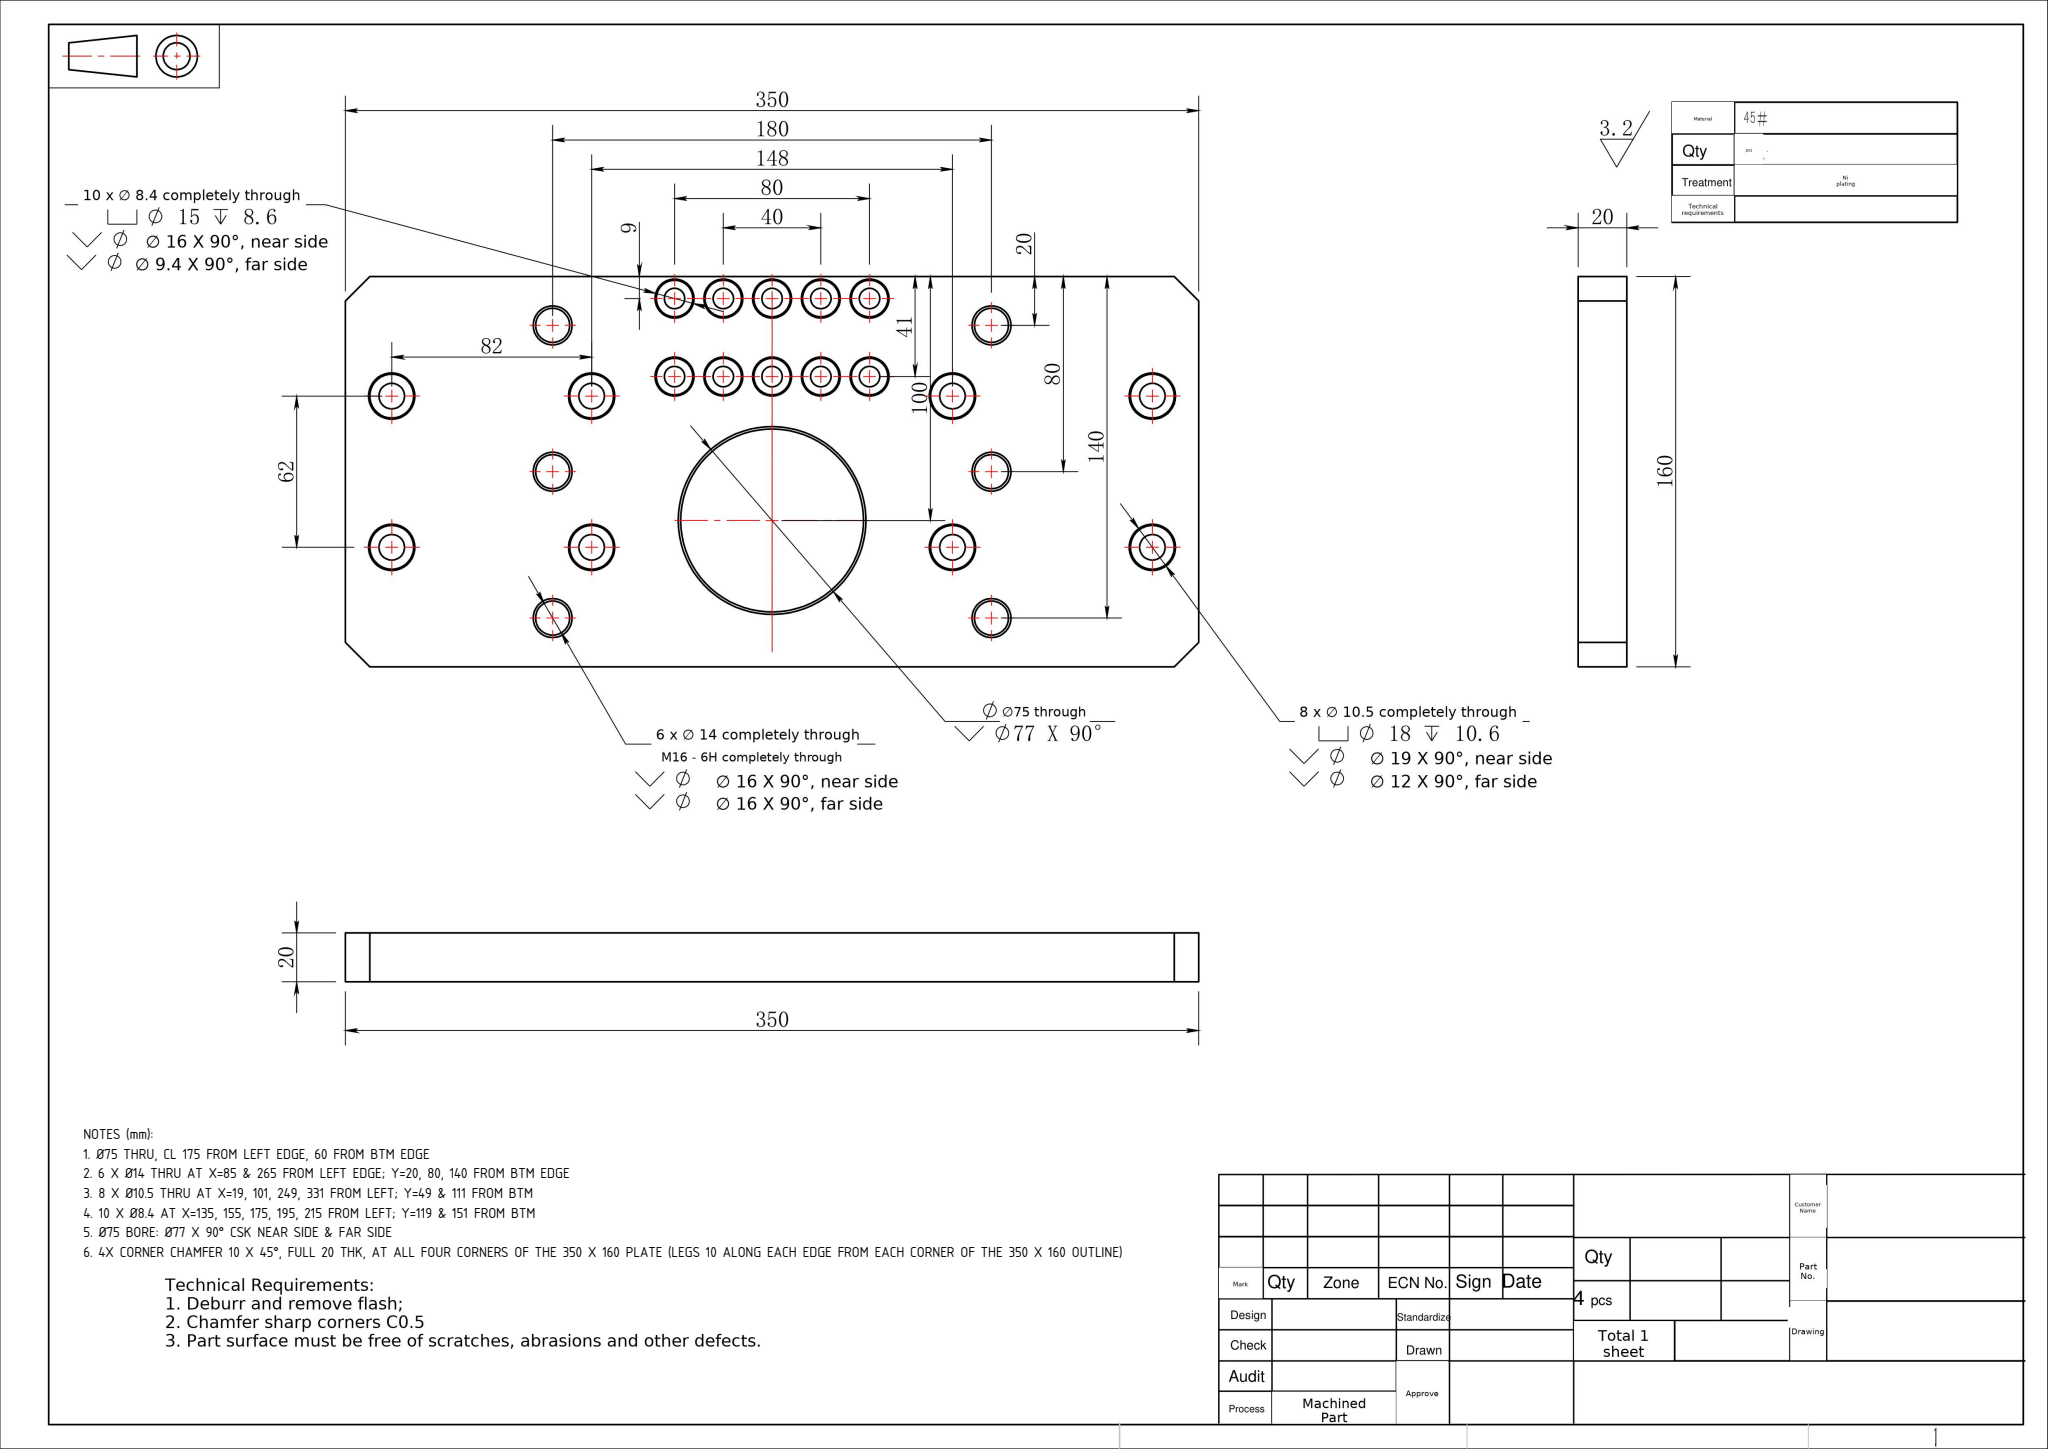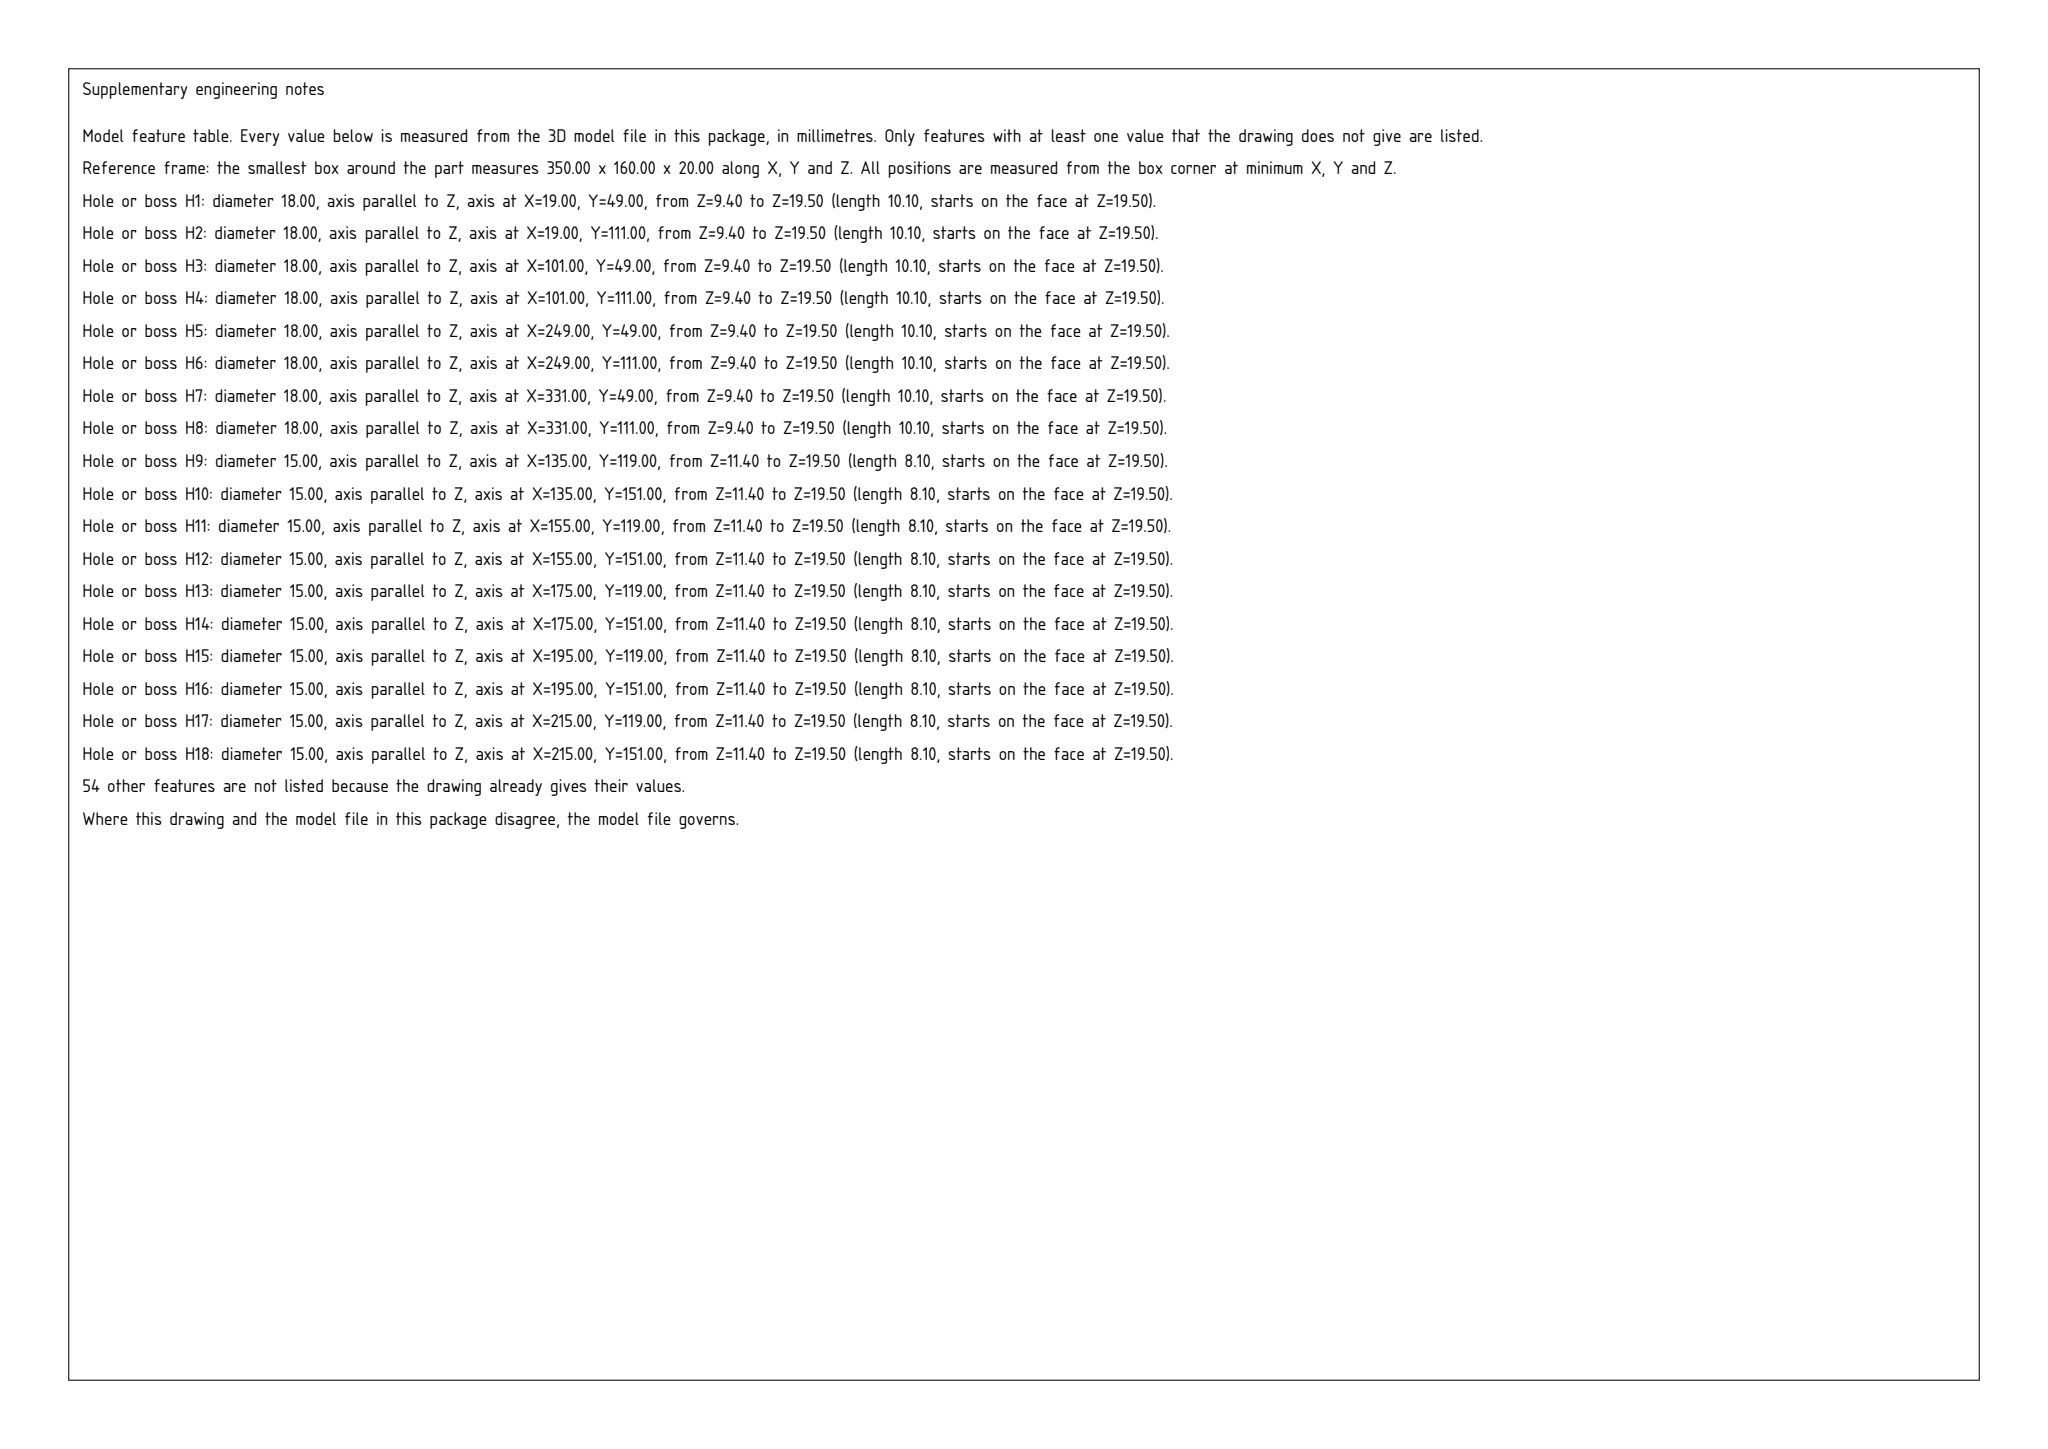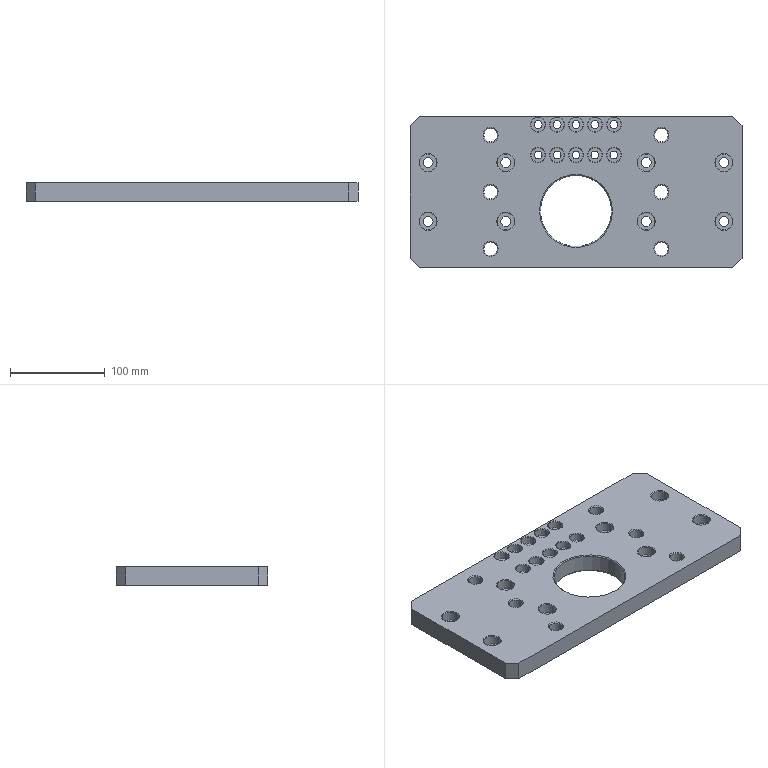Part | SolidWorks | mm | 1 solid | 214 faces | box 350 x 160 x 20 mm | volume 958820 mm3 | cone 100 | cylinder 86 | plane 28 | commonest cylinder face diameters 15 x20 8.4 x20 18 x16 10.5 x16 14 x12 75 x2
Drawing notes:
Ø75 THRU, CL 175 FROM LEFT EDGE, 60 FROM BTM EDGE | from the solid: Ø75 cylinder axis at [175.0, 60.0], bbox 350x160x20
6 X Ø14 THRU AT X=85 & 265 FROM LEFT EDGE; Y=20, 80, 140 FROM BTM EDGE | from the solid: Ø14 cylinders at x=85,265 and y=20,80,140
8 X Ø10.5 THRU AT X=19, 101, 249, 331 FROM LEFT; Y=49 & 111 FROM BTM | from the solid: Ø10.5 cylinders at x=19,101,249,331 and y=49,111
10 X Ø8.4 AT X=135, 155, 175, 195, 215 FROM LEFT; Y=119 & 151 FROM BTM | from the solid: Ø8.4 cylinders at x=135,155,175,195,215 and y=119,151
Ø75 BORE: Ø77 X 90° CSK NEAR SIDE & FAR SIDE | from the solid: Ø75 thru bore at (175,60); 90° cones ref Ø77 and Ø75 at both z faces (2 cones, one per face), csk depth (77-75)/2 = 1
4X CORNER CHAMFER 10 X 45°, FULL 20 THK, AT ALL FOUR CORNERS OF THE 350 X 160 PLATE (LEGS 10 ALONG EACH EDGE FROM EACH CORNER OF THE 350 X 160 OUTLINE) | from the solid: inclined_planes: 4X angle_to_xyz_axes [45,45,90], size [10,10,20], at bbox_from [0,0,0], [0,150,0], [340,0,0], [340,150,0]; axis_planes x=0 and x=350 extent y 10..150, y=0 and y=160 extent x 10..340